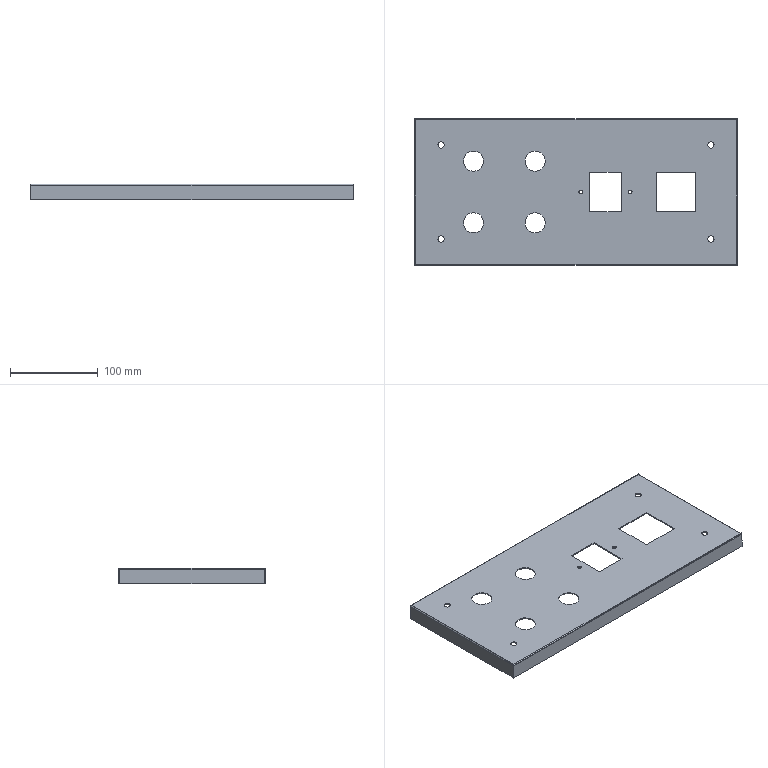Component | SolidWorks | FrontPanel-1 | 1 solid | 70 faces | volume 87998 mm3 | plane 42 | cylinder 28 | commonest cylinder face diameters 7 x8 23 x8 4.5 x4 2.6 x4 0.2 x4